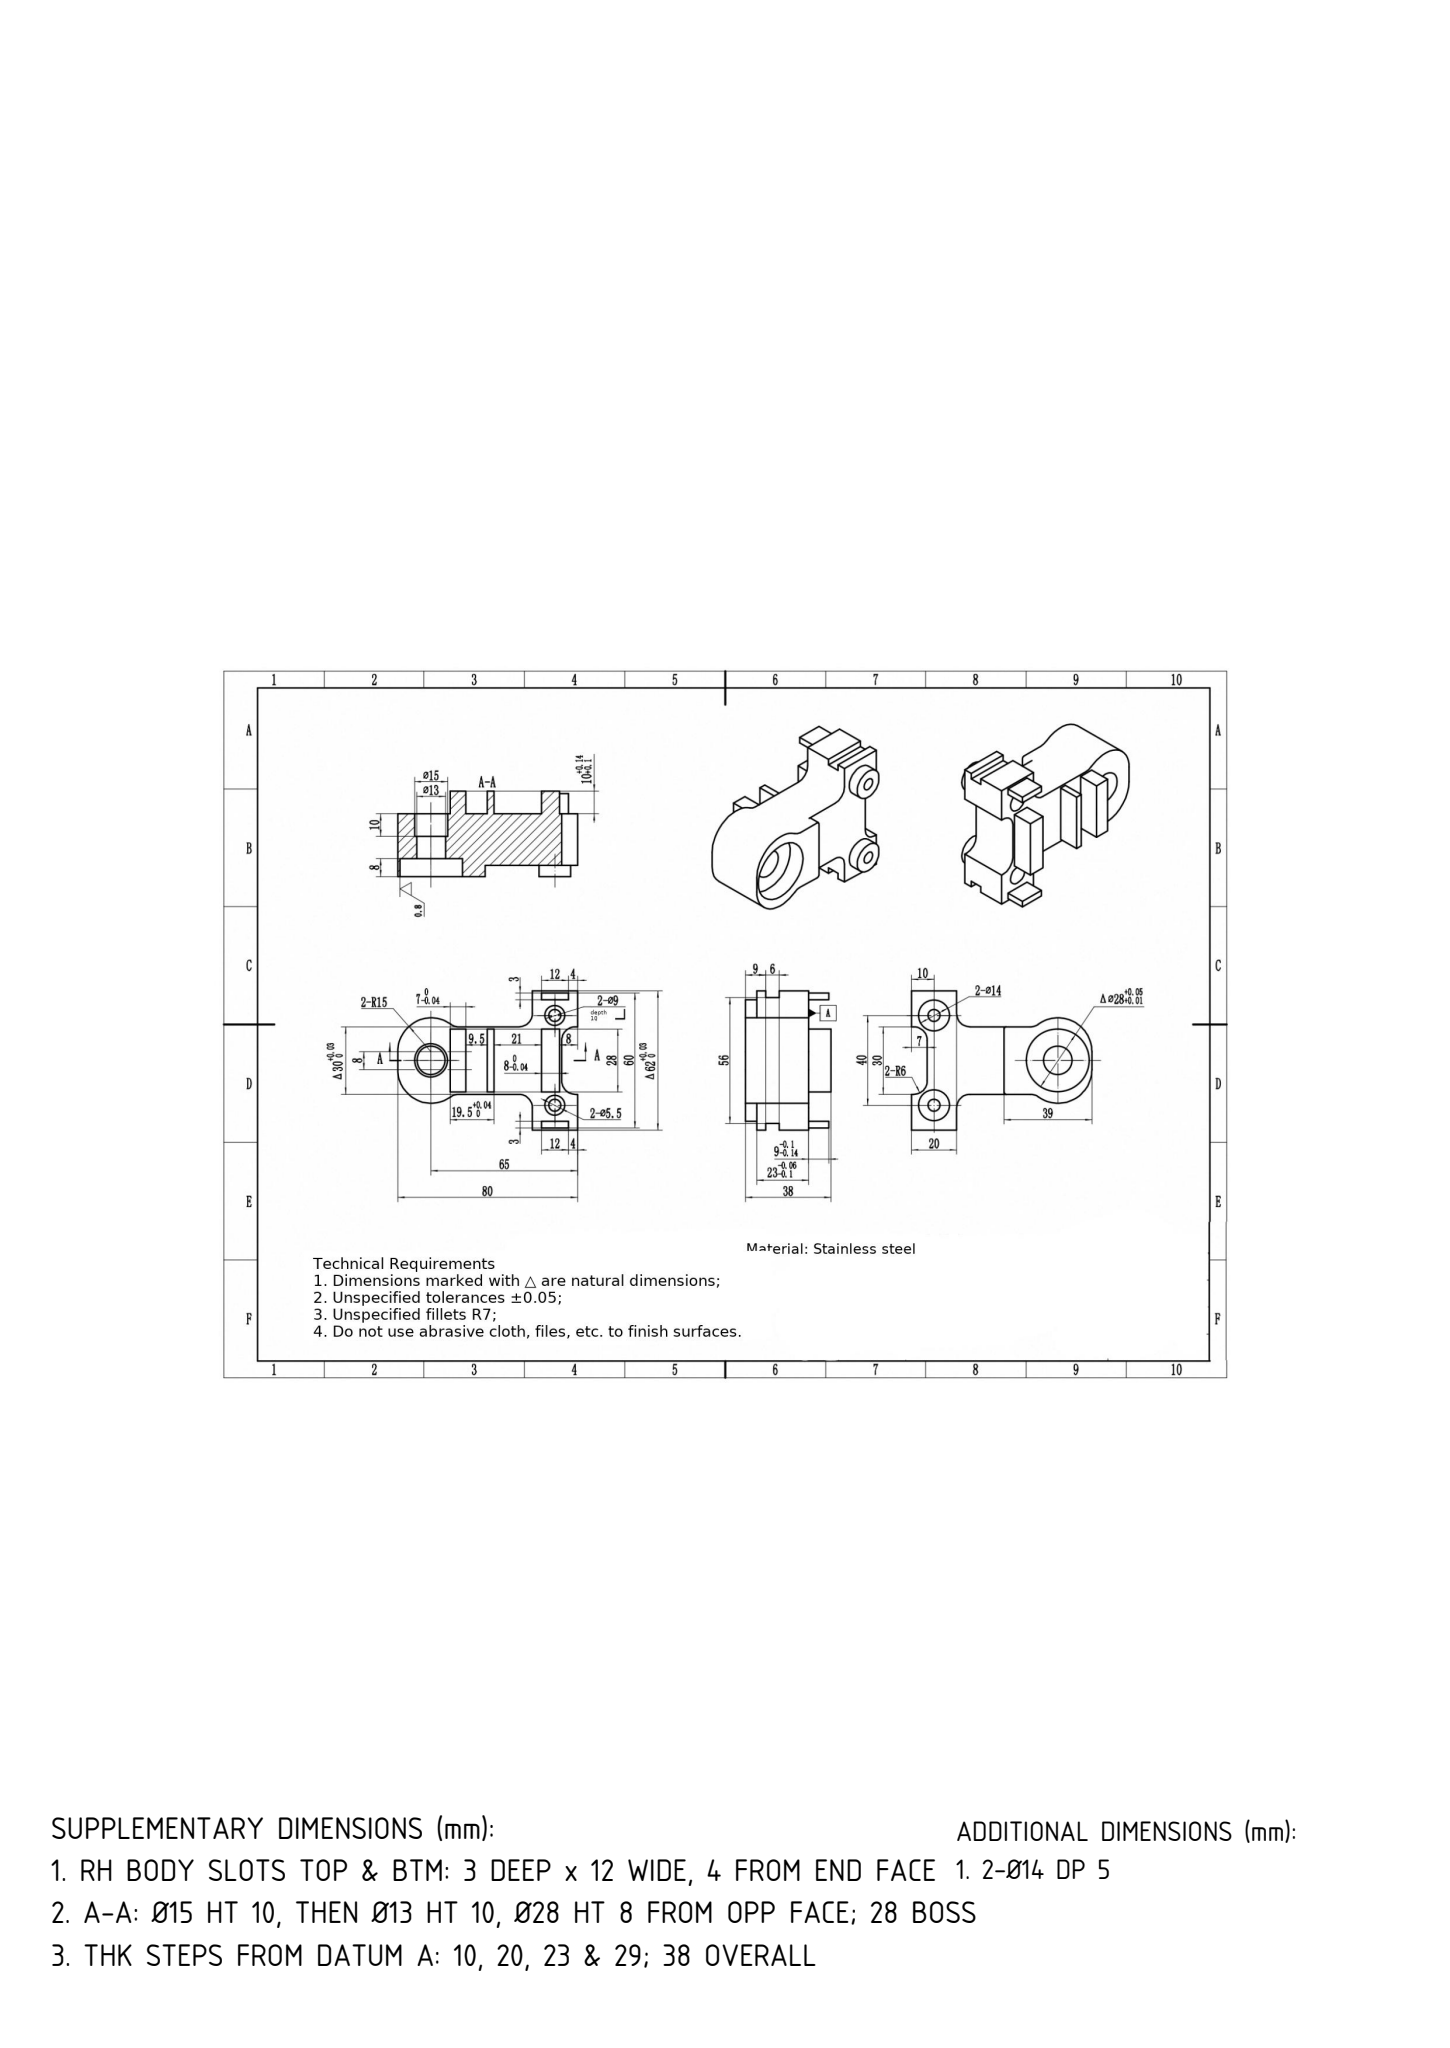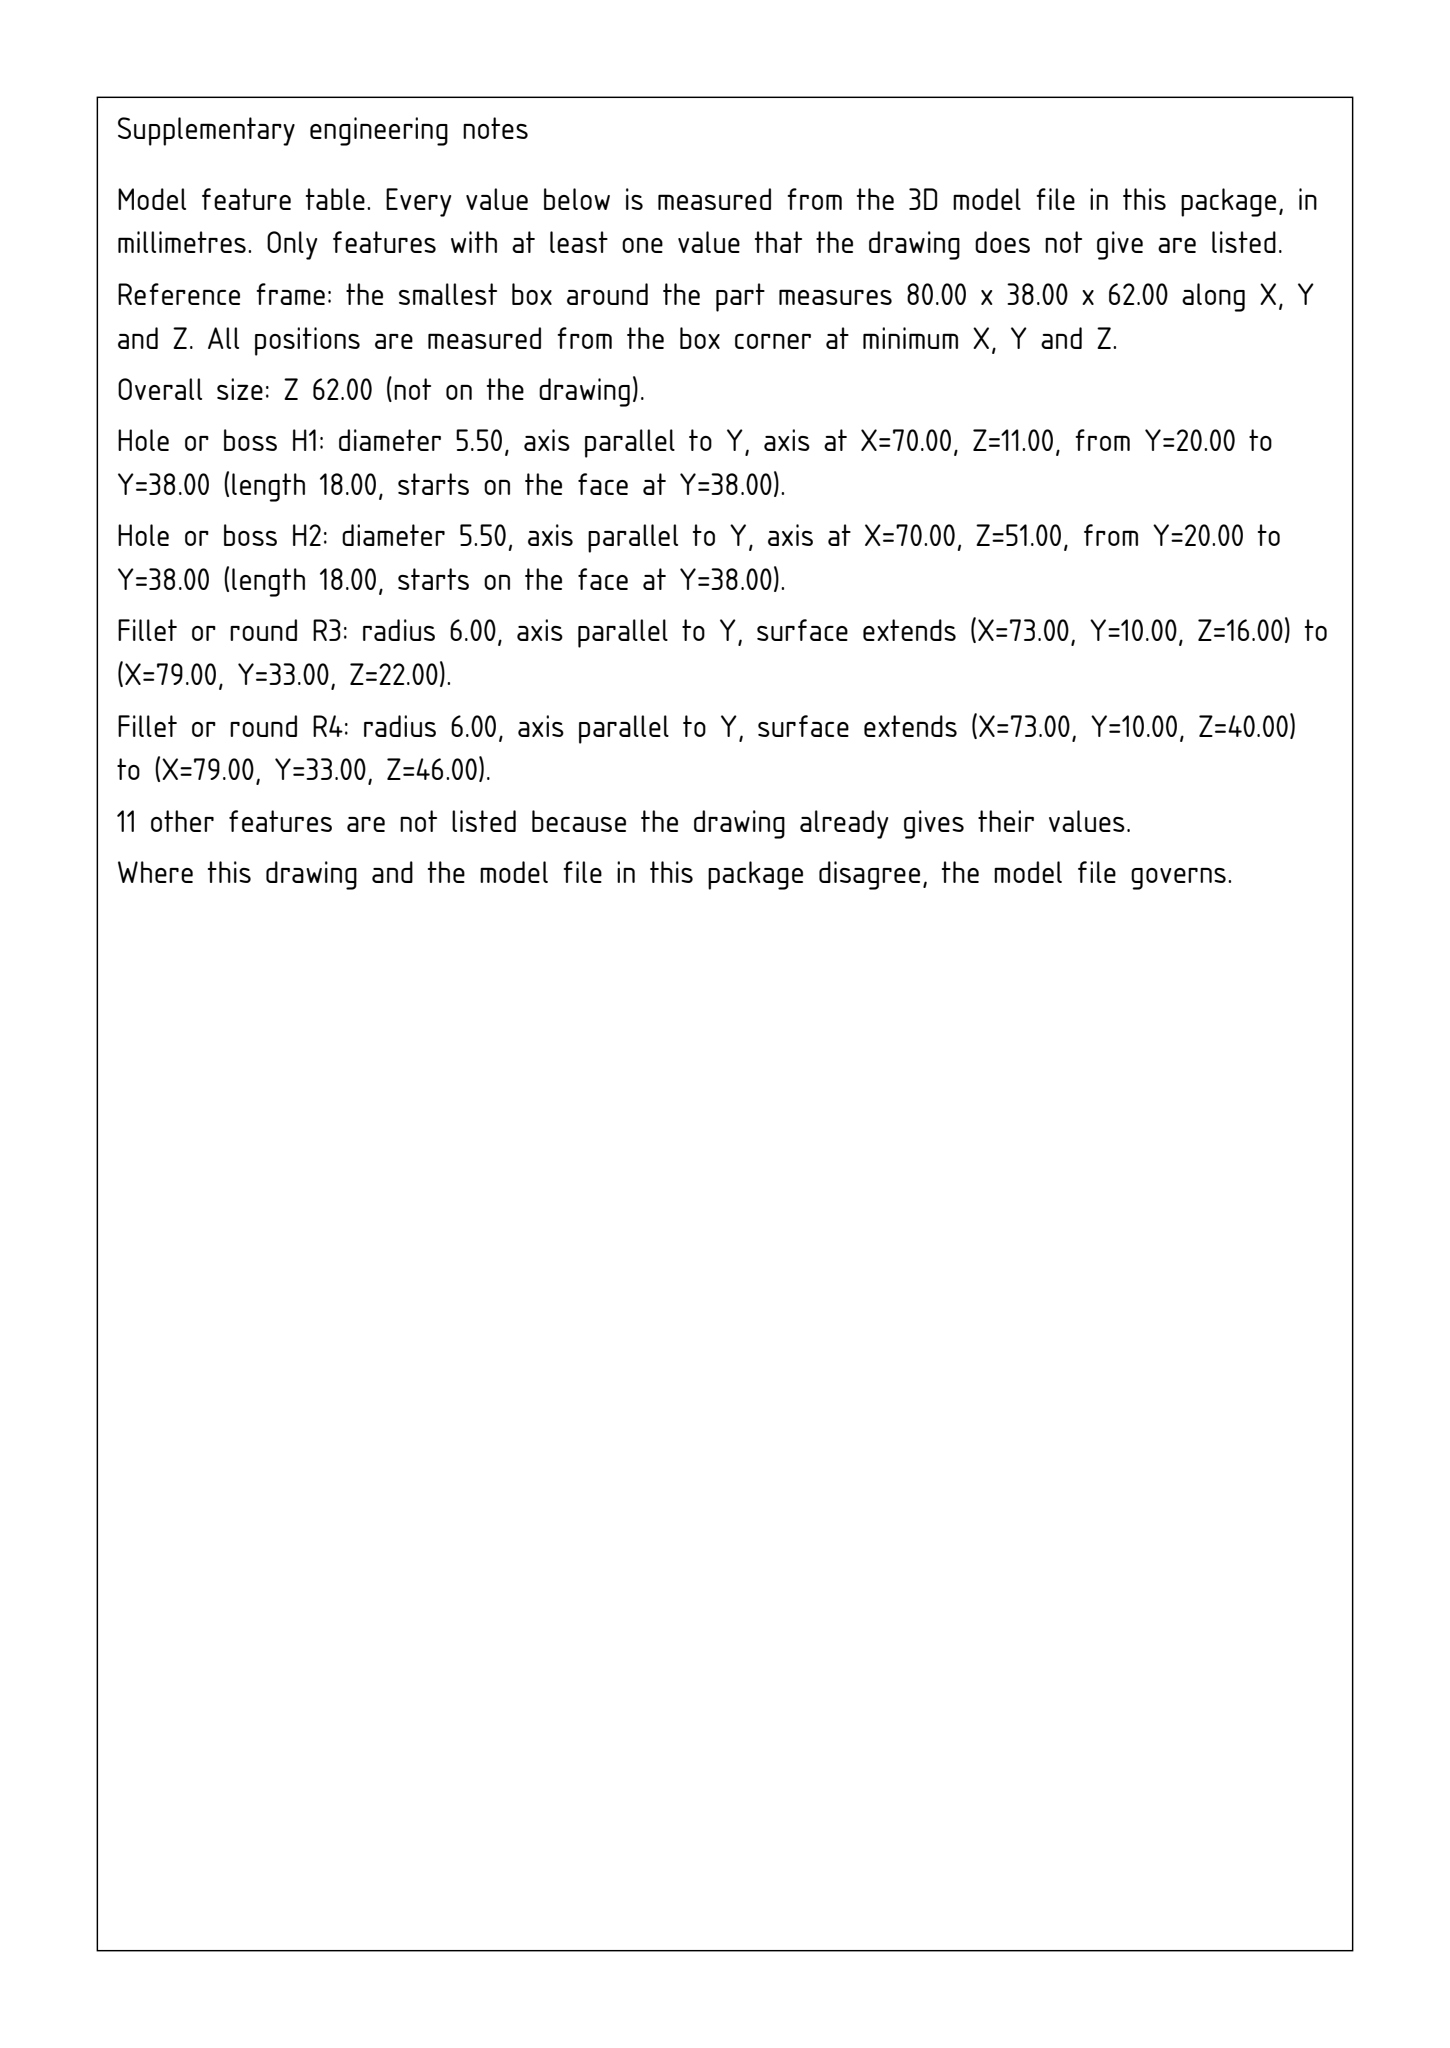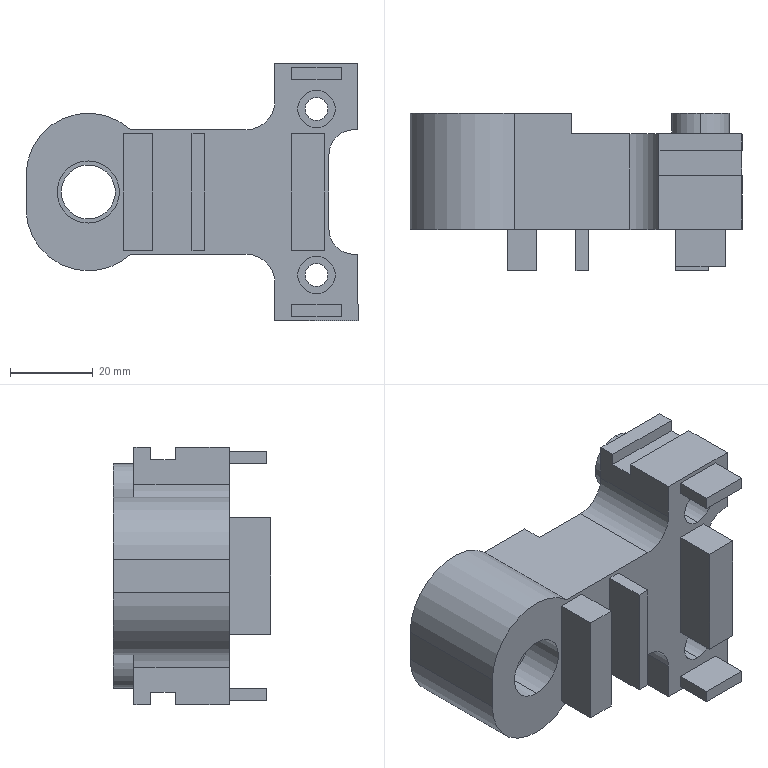Part | SolidWorks | mm | 1 solid | 80 faces | box 80 x 38 x 62 mm | volume 70363 mm3 | plane 55 | cylinder 25 | commonest cylinder face diameters 14 x6 9 x4 5.5 x4 30 x3 15 x2 28 x2 13 x2 12 x2
build123d program:
from build123d import *

# Parameters (mm, degrees)
SKETCH1_R           = 6.5
BOSS_EXTRUDE1_DEPTH = 23
SKETCH2_R           = 6.5
BOSS_EXTRUDE2_DEPTH = 5
SKETCH3_R           = 14
CUT_EXTRUDE1_DEPTH  = 8
SKETCH4_R           = 7.5
CUT_EXTRUDE2_DEPTH  = 10
SKETCH5_R           = 7
BOSS_EXTRUDE3_DEPTH = 5
SKETCH6_3_W         = 7
SKETCH6_3_H         = 28
SKETCH6_3_W_2       = 3
SKETCH6_3_W_3       = 8
BOSS_EXTRUDE4_DEPTH = 10
SKETCH6_3_2_W       = 12
SKETCH6_3_2_H       = 3
BOSS_EXTRUDE5_DEPTH = 9
SKETCH8_W           = 3
SKETCH8_H           = 6
CUT_EXTRUDE3_DEPTH  = 91.25
HOLE1_D             = 5.5
HOLE1_DEPTH         = 100
HOLE1_CBORE_D       = 9
HOLE1_CBORE_DEPTH   = 10


with BuildPart() as part:
    # Sketch1 → Boss-Extrude1 (new body)
    with BuildSketch(Plane(origin=(0, 0, 0), x_dir=(1, 0, 0), z_dir=(0, 1, 0))):
        with BuildLine():
            Line((-15, 4), (-15, -4))
            ThreePointArc((-15, -4), (-6.001, -17.747), (10.198, -15))
            Line((10.198, -15), (38, -15))
            ThreePointArc((38, -15), (42.95, -17.05), (45, -22))
            Line((45, -22), (45, -31))
            Line((45, -31), (65, -31))
            Line((65, -31), (65, -15))
            Line((65, -15), (64, -15))
            ThreePointArc((64, -15), (59.757, -13.243), (58, -9))
            Line((58, -9), (58, 9))
            ThreePointArc((58, 9), (59.757, 13.243), (64, 15))
            Line((64, 15), (65, 15))
            Line((65, 15), (65, 31))
            Line((65, 31), (45, 31))
            Line((45, 31), (45, 22))
            ThreePointArc((45, 22), (42.95, 17.05), (38, 15))
            Line((38, 15), (10.198, 15))
            ThreePointArc((10.198, 15), (-6.001, 17.747), (-15, 4))
        make_face()
        with Locations(Location((0, 0, 0), (0, 0, 270))):
            Circle(SKETCH1_R, mode=Mode.SUBTRACT)
    extrude(amount=BOSS_EXTRUDE1_DEPTH)

    # Sketch2 → Boss-Extrude2 (add)
    with BuildSketch(Plane(origin=(0, 23, 0), x_dir=(1, 0, 0), z_dir=(0, 1, 0))):
        with BuildLine():
            Line((24, 15), (24, -15))
            Line((24, -15), (10.198, -15))
            ThreePointArc((10.198, -15), (-6.001, -17.747), (-15, -4))
            Line((-15, -4), (-15, 4))
            ThreePointArc((-15, 4), (-6.001, 17.747), (10.198, 15))
            Line((10.198, 15), (24, 15))
        make_face()
        with Locations(Location((0, 0, 0), (0, 0, 270))):
            Circle(SKETCH2_R, mode=Mode.SUBTRACT)
    extrude(amount=BOSS_EXTRUDE2_DEPTH)

    # Sketch3 → Cut-Extrude1 (cut)
    with BuildSketch(Plane(origin=(0, 28, 0), x_dir=(1, 0, 0), z_dir=(0, 1, 0))):
        with Locations(Location((0, 0, 0), (0, 0, 270))):
            Circle(SKETCH3_R)
    extrude(amount=-CUT_EXTRUDE1_DEPTH, mode=Mode.SUBTRACT)

    # Sketch4 → Cut-Extrude2 (cut)
    with BuildSketch(Plane.XZ):
        with Locations(Location((0, 0, 0), (0, 0, 270))):
            Circle(SKETCH4_R)
    extrude(amount=-CUT_EXTRUDE2_DEPTH, mode=Mode.SUBTRACT)

    # Sketch5 → Boss-Extrude3 (add)
    with BuildSketch(Plane(origin=(0, 23, 0), x_dir=(1, 0, 0), z_dir=(0, 1, 0))):
        with Locations(Location((55, 20, 0), (0, 0, 270))):
            Circle(SKETCH5_R)
        with Locations(Location((55, -20, 0), (0, 0, 90))):
            Circle(SKETCH5_R)
    extrude(amount=BOSS_EXTRUDE3_DEPTH)

    # Sketch6_3 → Boss-Extrude4 (add)
    with BuildSketch(Plane.XZ):
        with Locations((12, 0)):
            Rectangle(SKETCH6_3_W, SKETCH6_3_H)
        with Locations((26.5, 0)):
            Rectangle(SKETCH6_3_W_2, SKETCH6_3_H)
        with Locations((53, 0)):
            Rectangle(SKETCH6_3_W_3, SKETCH6_3_H)
    extrude(amount=BOSS_EXTRUDE4_DEPTH)

    # Sketch6_3 2 → Boss-Extrude5 (add)
    with BuildSketch(Plane.XZ):
        with Locations((55, -28.5)):
            Rectangle(SKETCH6_3_2_W, SKETCH6_3_2_H)
        with Locations((55, 28.5)):
            Rectangle(SKETCH6_3_2_W, SKETCH6_3_2_H)
    extrude(amount=BOSS_EXTRUDE5_DEPTH)

    # Sketch8 → Cut-Extrude3 (cut, through all)
    with BuildSketch(Plane(origin=(65, 0, 0), x_dir=(0, 0, -1), z_dir=(1, 0, 0))):
        with Locations((29.5, 16)):
            Rectangle(SKETCH8_W, SKETCH8_H)
        with Locations((-29.5, 16)):
            Rectangle(SKETCH8_W, SKETCH8_H)
    extrude(amount=-CUT_EXTRUDE3_DEPTH, mode=Mode.SUBTRACT)

    # Hole1
    with Locations(Plane.XZ):
        with Locations((55, -20), (55, 20)):
            CounterBoreHole(HOLE1_D / 2, HOLE1_CBORE_D / 2, HOLE1_CBORE_DEPTH, depth=HOLE1_DEPTH)


solid = part.part